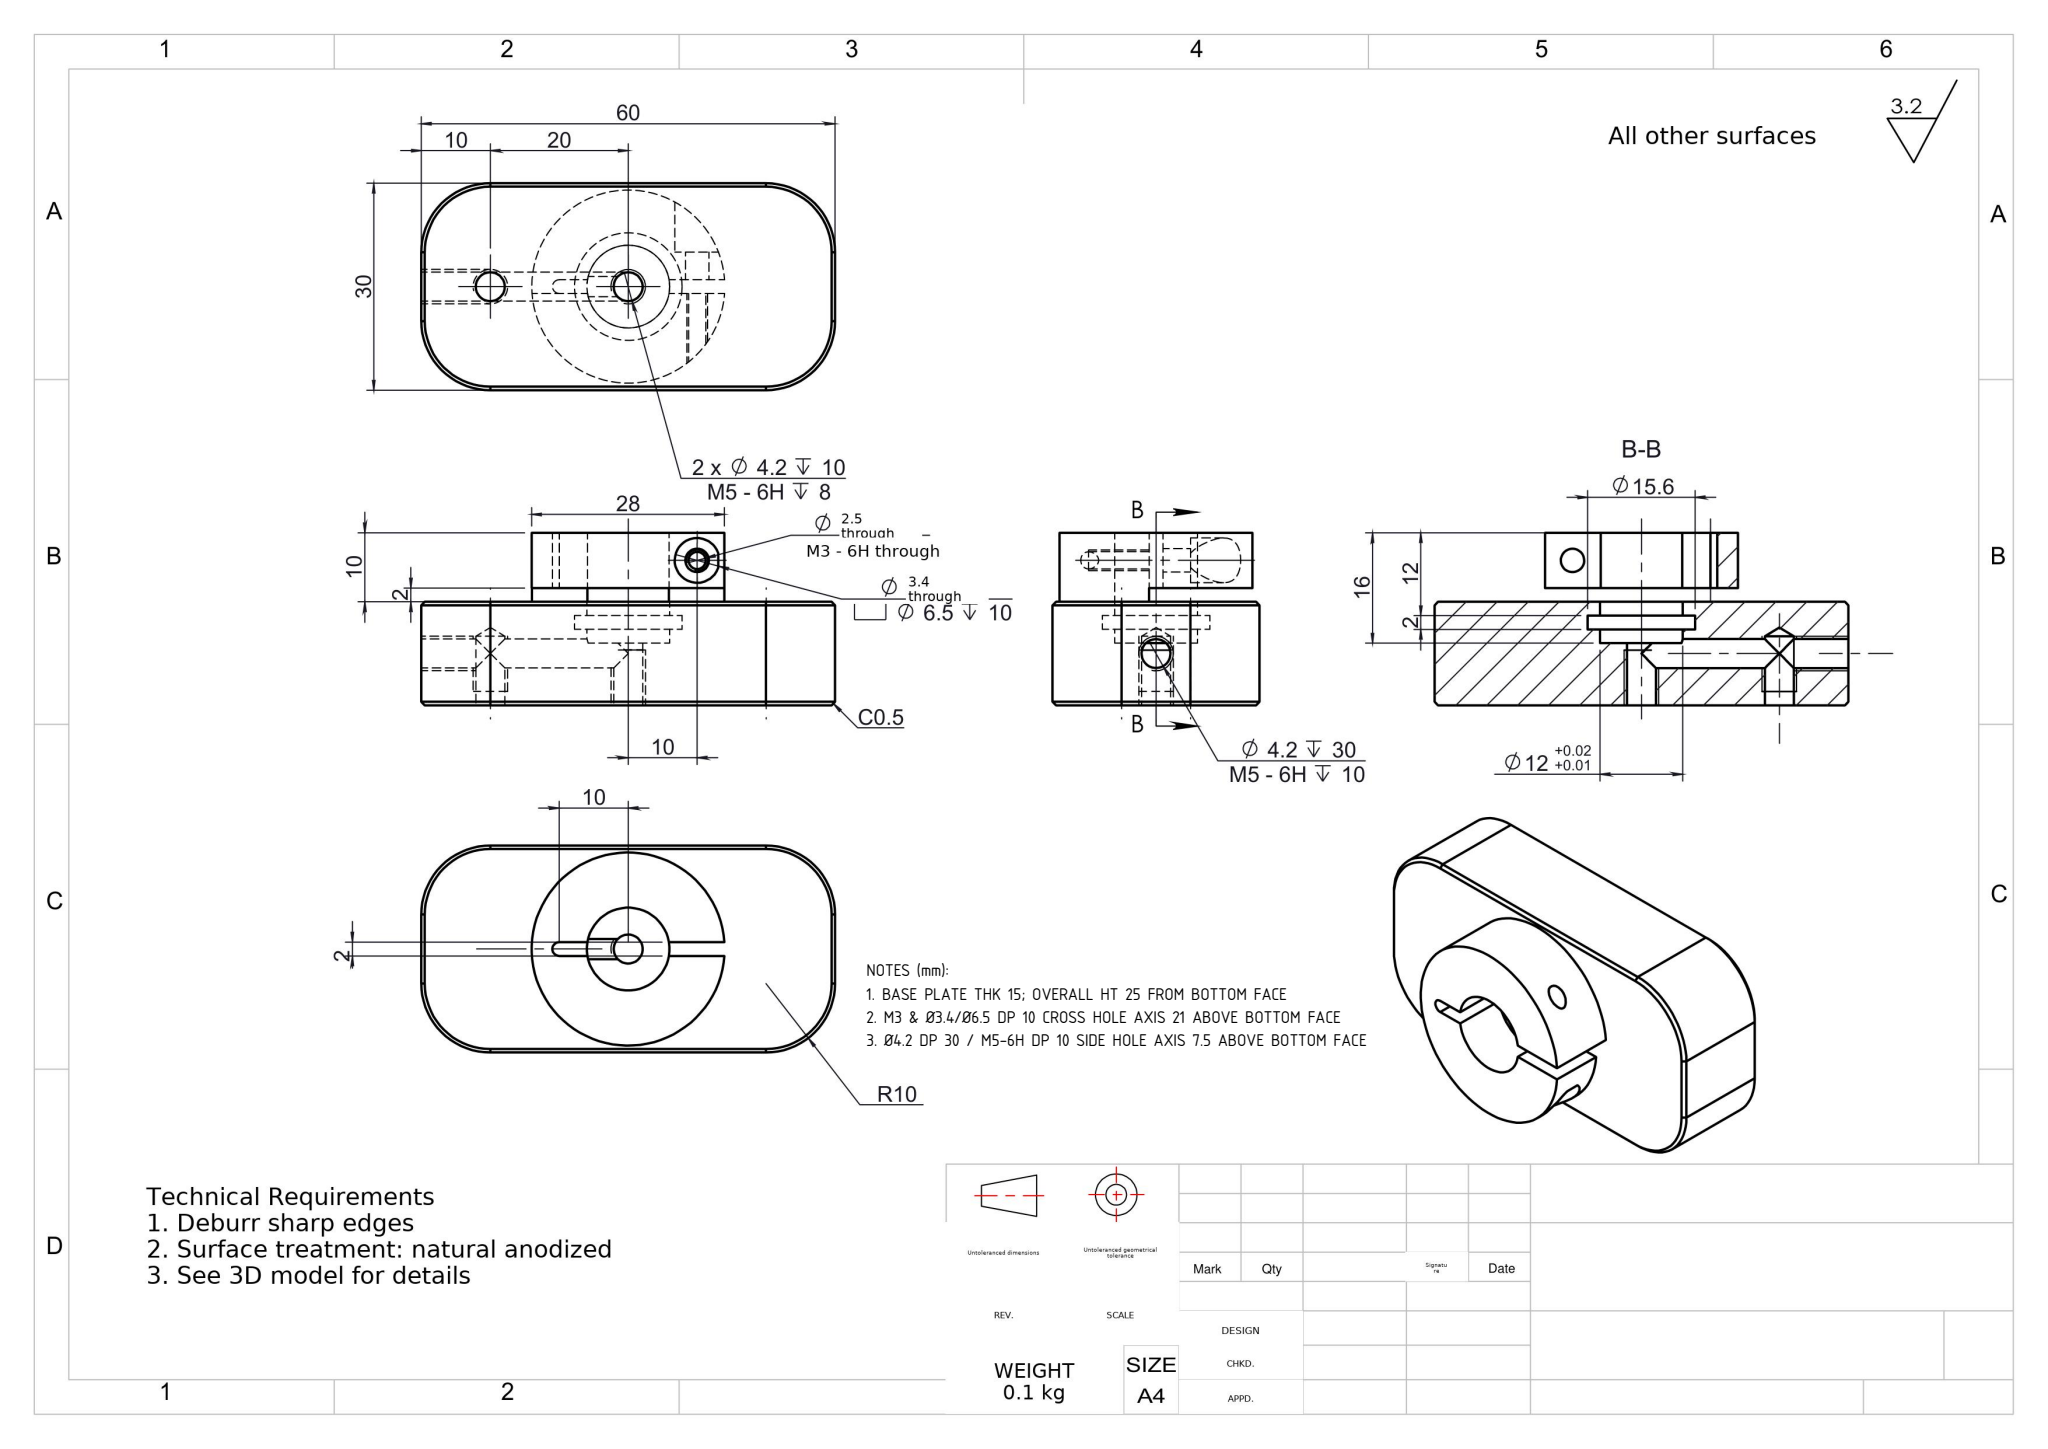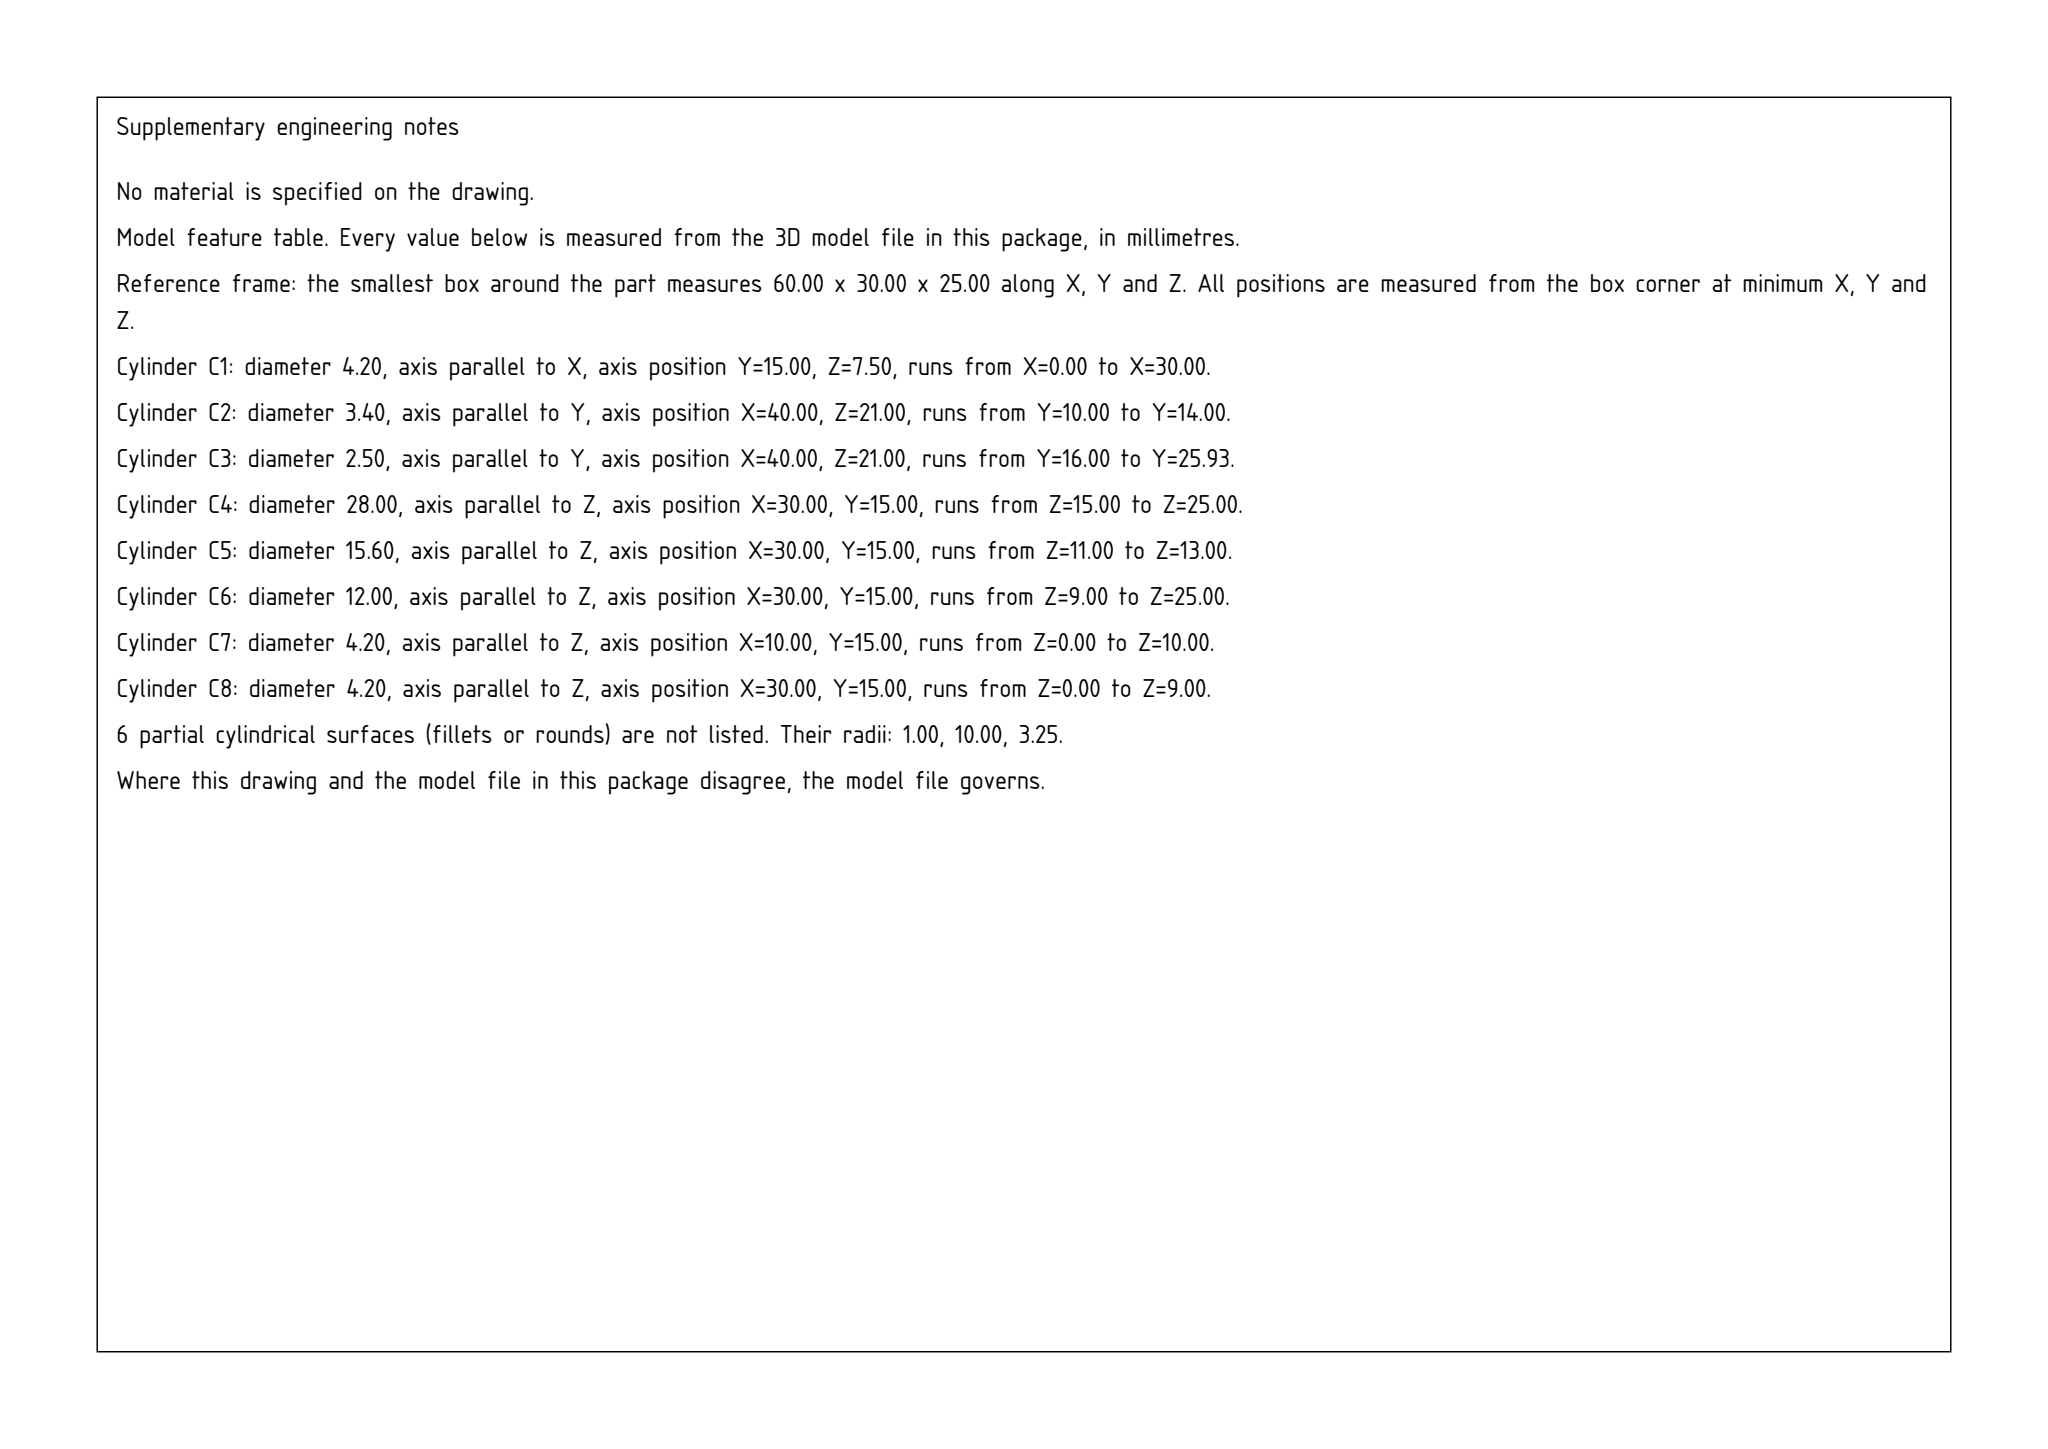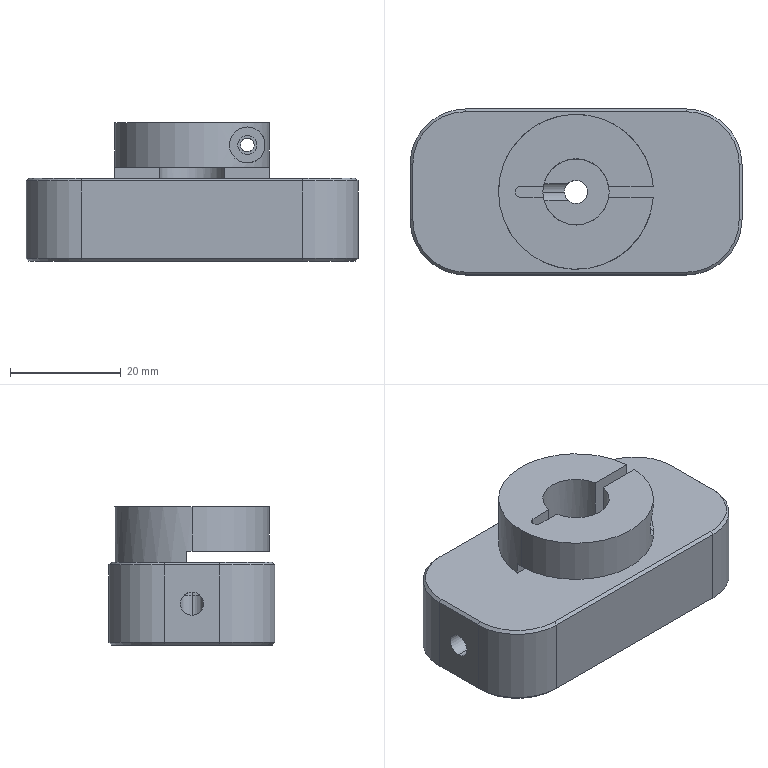Part | SolidWorks | mm | 1 solid | 66 faces | box 60 x 30 x 25 mm | volume 28290 mm3 | cylinder 32 | plane 24 | cone 10 | commonest cylinder face diameters 4.2 x10 12 x5 20 x4 6.5 x3 2.5 x2 3.4 x2 2 x2 15.6 x2
Drawing notes:
BASE PLATE THK 15; OVERALL HT 25 FROM BOTTOM FACE | from the solid: z-planes at 0, 15 (plate top) and 25 (boss top); bbox z=25
M3 & Ø3.4/Ø6.5 DP 10 CROSS HOLE AXIS 21 ABOVE BOTTOM FACE | from the solid: cylinders dia 2.5/3.4/6.5 axis y at z=21.0
Ø4.2 DP 30 / M5-6H DP 10 SIDE HOLE AXIS 7.5 ABOVE BOTTOM FACE | from the solid: hole dia 4.2 axis x at [y=15.0, z=7.5], from 0 to 30